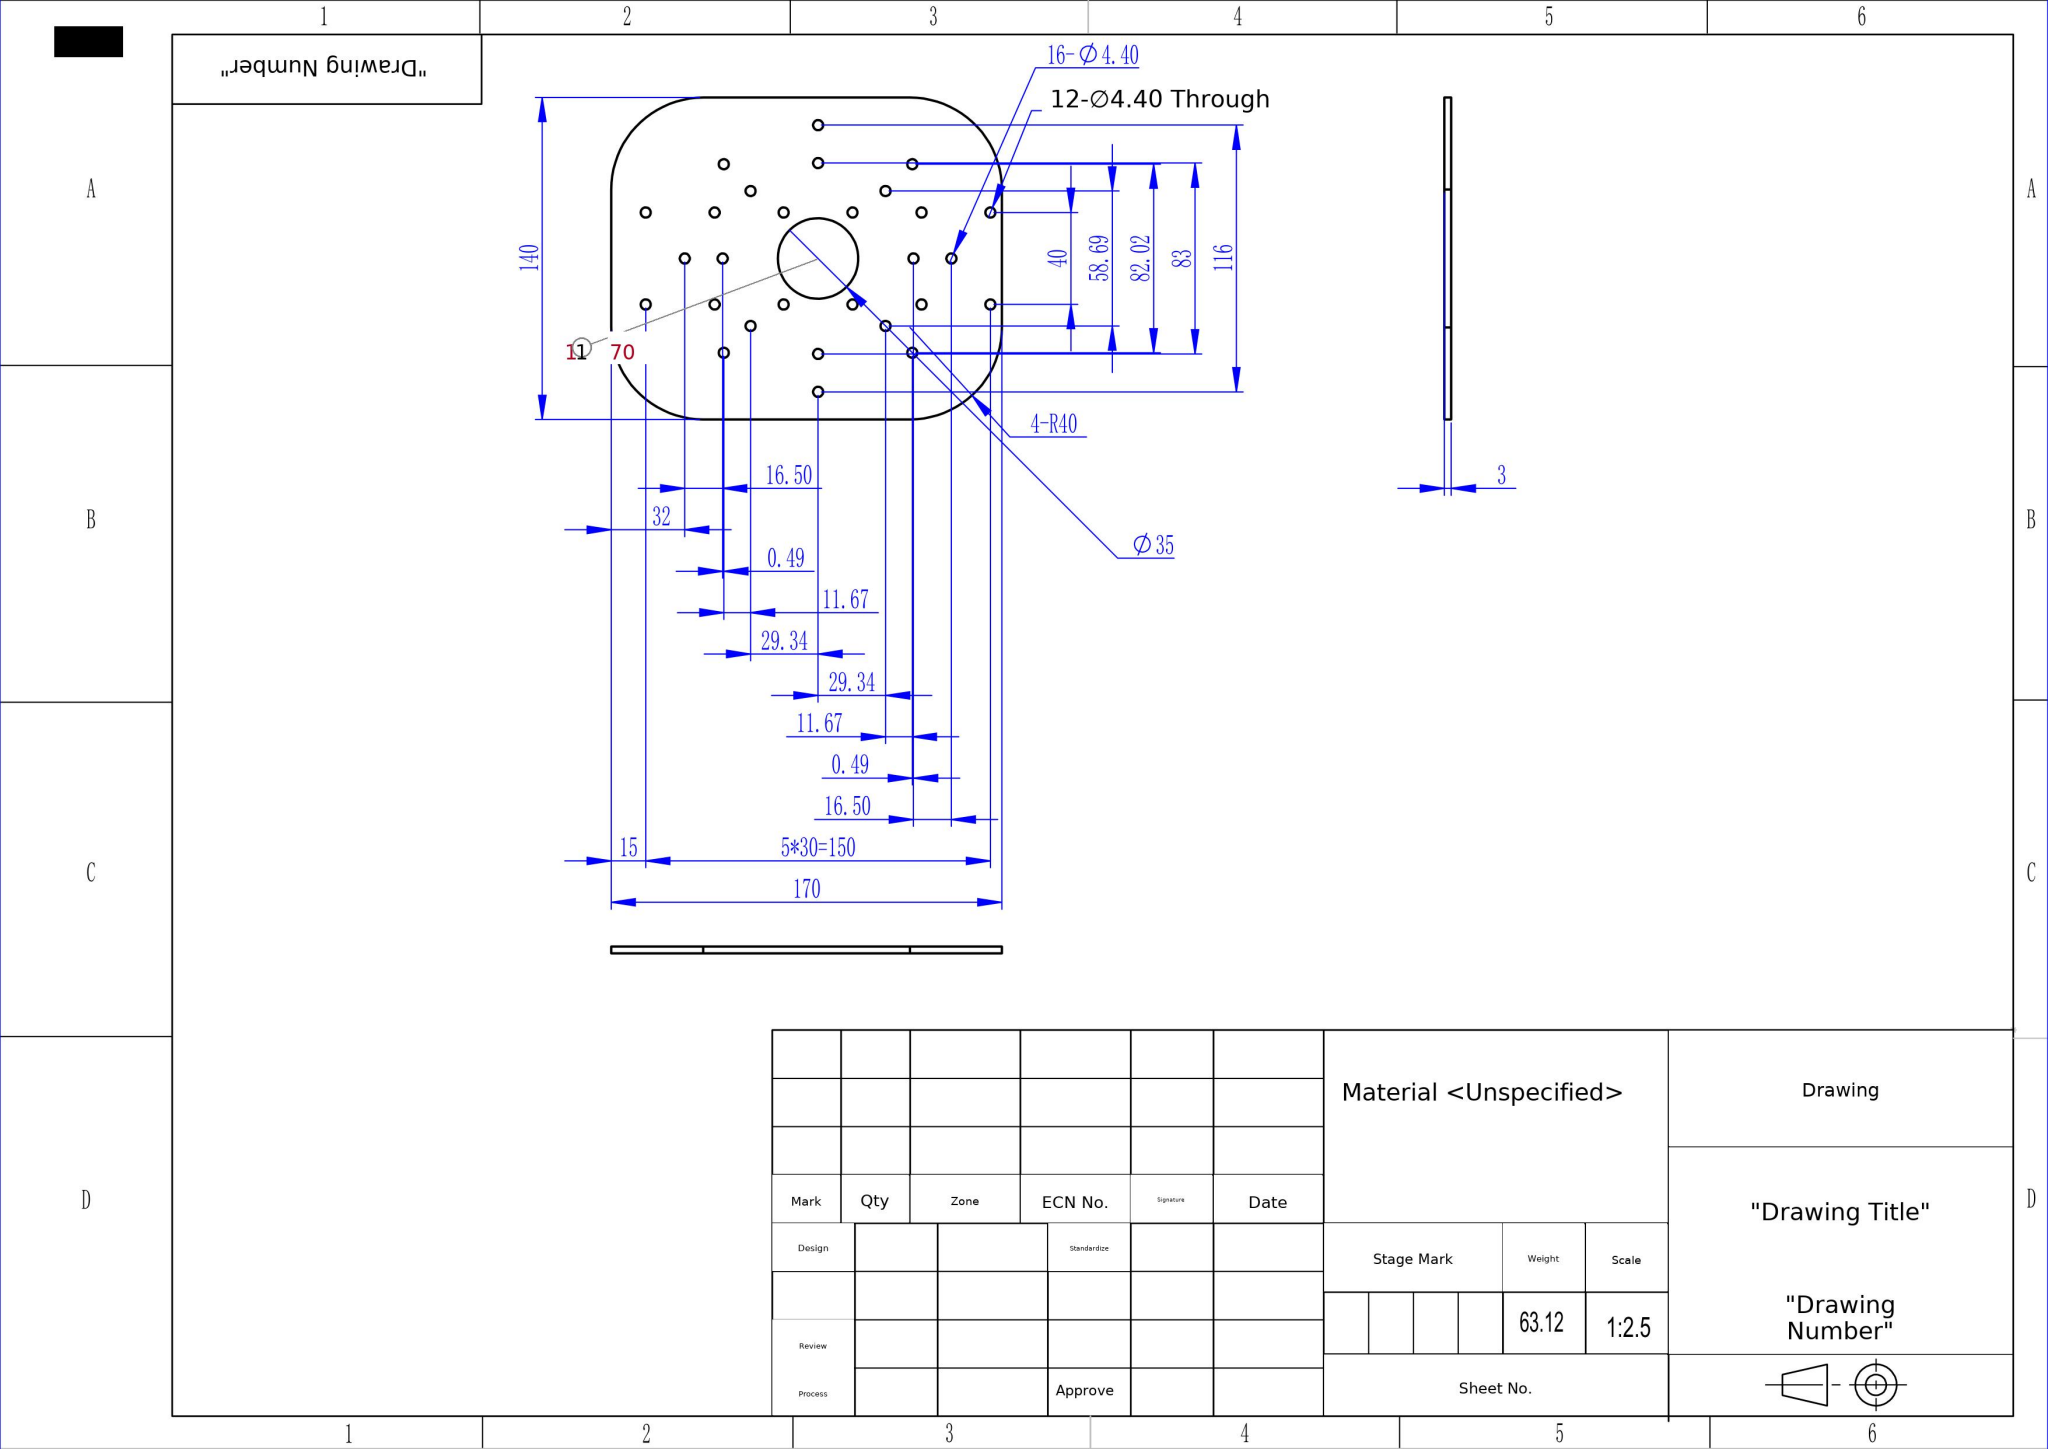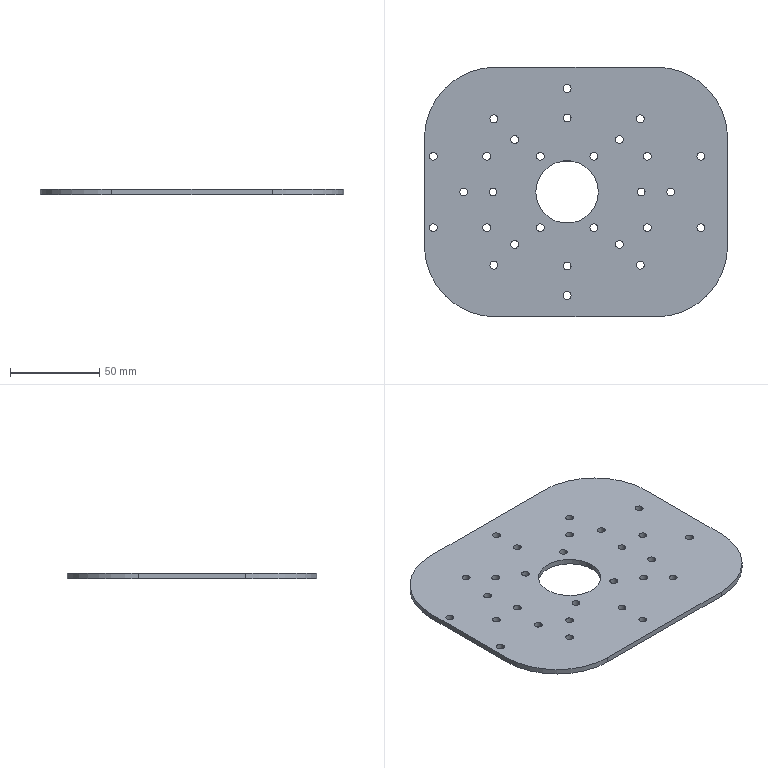Part | SolidWorks | mm | 1 solid | 68 faces | box 170 x 140 x 3 mm | volume 63116 mm3 | cylinder 62 | plane 6 | commonest cylinder face diameters 4.4 x56 80 x4 35 x2
build123d program:
from build123d import *

# Parameters (mm, degrees)
SKETCH1_R           = 2.2
SKETCH1_R_2         = 17.5
BOSS_EXTRUDE1_DEPTH = 3
SKETCH2_R           = 2.2
CUT_EXTRUDE1_DEPTH  = 115.057
FILLET1_R           = 40


with BuildPart() as part:
    # Sketch1 → Boss-Extrude1 (new body)
    with BuildSketch(Plane.XY):
        Polygon((0, 70), (90, 70), (90, -70), (0, -70), (-80, -70), (-80, 70), align=None)
        with Locations((41.5, 0)):
            Circle(SKETCH1_R, mode=Mode.SUBTRACT)
        with Locations((-58, 0)):
            Circle(SKETCH1_R, mode=Mode.SUBTRACT)
        with Locations((58, 0)):
            Circle(SKETCH1_R, mode=Mode.SUBTRACT)
        with Locations((0, -58)):
            Circle(SKETCH1_R, mode=Mode.SUBTRACT)
        with Locations((41.012, -41.012)):
            Circle(SKETCH1_R, mode=Mode.SUBTRACT)
        with Locations((-41.012, -41.012)):
            Circle(SKETCH1_R, mode=Mode.SUBTRACT)
        with Locations((41.012, 41.012)):
            Circle(SKETCH1_R, mode=Mode.SUBTRACT)
        with Locations((-41.012, 41.012)):
            Circle(SKETCH1_R, mode=Mode.SUBTRACT)
        with Locations((0, 58)):
            Circle(SKETCH1_R, mode=Mode.SUBTRACT)
        Circle(SKETCH1_R_2, mode=Mode.SUBTRACT)
        with Locations((29.345, -29.345)):
            Circle(SKETCH1_R, mode=Mode.SUBTRACT)
        with Locations((0, -41.5)):
            Circle(SKETCH1_R, mode=Mode.SUBTRACT)
        with Locations((-29.345, -29.345)):
            Circle(SKETCH1_R, mode=Mode.SUBTRACT)
        with Locations((-41.5, 0)):
            Circle(SKETCH1_R, mode=Mode.SUBTRACT)
        with Locations((-29.345, 29.345)):
            Circle(SKETCH1_R, mode=Mode.SUBTRACT)
        with Locations((0, 41.5)):
            Circle(SKETCH1_R, mode=Mode.SUBTRACT)
        with Locations((29.345, 29.345)):
            Circle(SKETCH1_R, mode=Mode.SUBTRACT)
    extrude(amount=BOSS_EXTRUDE1_DEPTH)

    # Sketch2 → Cut-Extrude1 (cut, through all)
    with BuildSketch(Plane.XY.offset(3)):
        with Locations((-75, 20)):
            Circle(SKETCH2_R)
        with Locations((-45, 20)):
            Circle(SKETCH2_R)
        with Locations((-15, 20)):
            Circle(SKETCH2_R)
        with Locations((15, 20)):
            Circle(SKETCH2_R)
        with Locations((45, 20)):
            Circle(SKETCH2_R)
        with Locations((75, 20)):
            Circle(SKETCH2_R)
        with Locations((-45, -20)):
            Circle(SKETCH2_R)
        with Locations((-15, -20)):
            Circle(SKETCH2_R)
        with Locations((15, -20)):
            Circle(SKETCH2_R)
        with Locations((45, -20)):
            Circle(SKETCH2_R)
        with Locations((75, -20)):
            Circle(SKETCH2_R)
        with Locations((-75, -20)):
            Circle(SKETCH2_R)
    extrude(amount=-CUT_EXTRUDE1_DEPTH, mode=Mode.SUBTRACT)

    # Fillet1
    fillet1_edges = [part.edges().sort_by_distance(p)[0] for p in [
        (90, 70, 1.5),
        (90, -70, 1.5),
        (-80, -70, 1.5),
        (-80, 70, 1.5),
    ]]
    fillet(fillet1_edges, radius=FILLET1_R)


solid = part.part